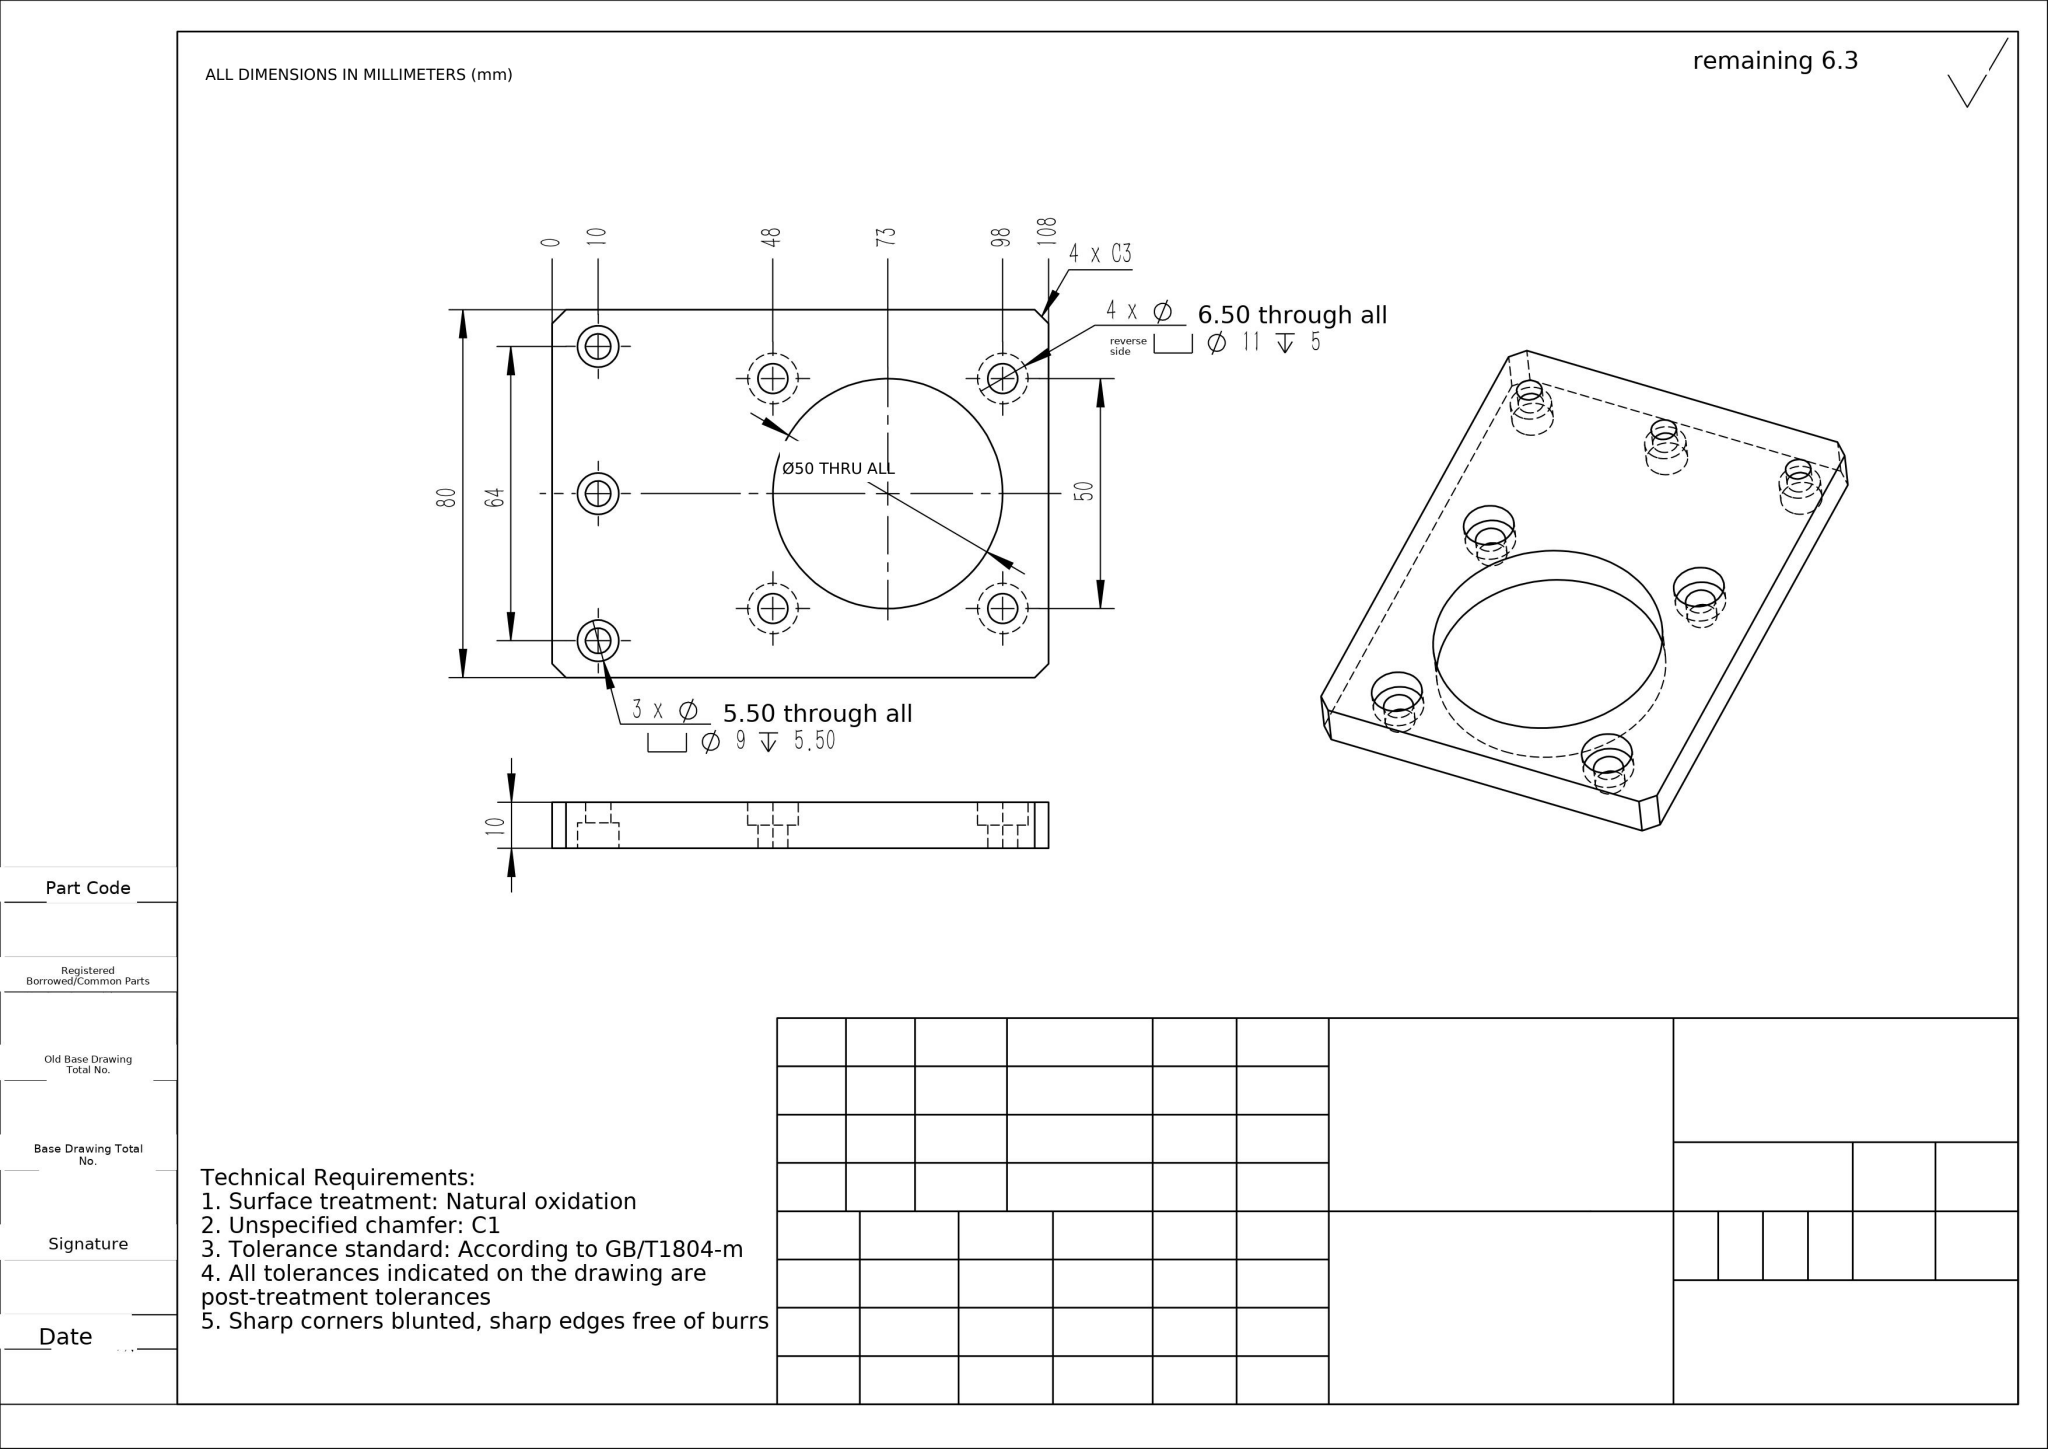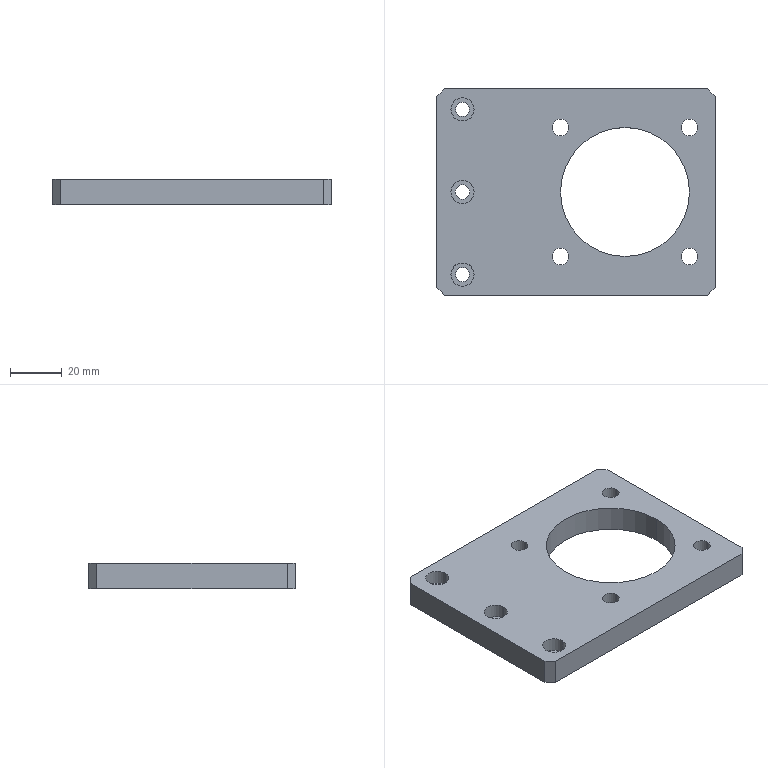Part | NX | mm | 1 solid | 47 faces | box 108 x 80 x 10 mm | volume 62650 mm3 | cylinder 30 | plane 17 | commonest cylinder face diameters 11 x8 6.5 x8 9 x6 5.5 x6 50 x2